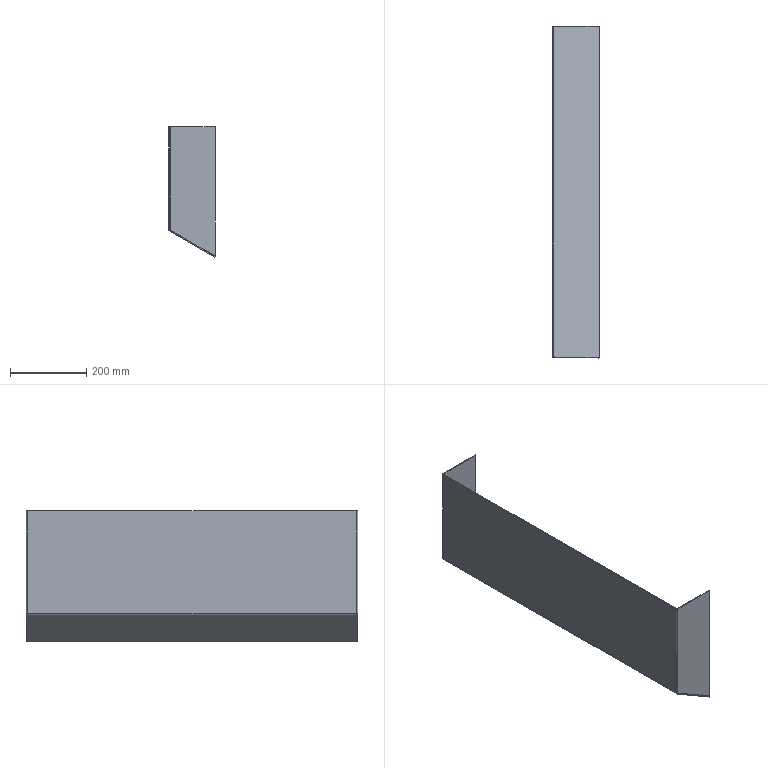Component | SolidWorks | AirInletVentAssembly-1_AirInletVentBaffle-5 | 1 solid | 32 faces | box 122 x 870 x 341.73 mm | volume 858235 mm3 | plane 24 | cylinder 6 | spline 2 | commonest cylinder face diameters 4 x3 8 x3 | material Plain Carbon Steel
STEP:
#1=CARTESIAN_POINT('',(96.744,7.148,50.154));
#2=VERTEX_POINT('',#1);
#3=CARTESIAN_POINT('',(96.744,41.085,50.154));
#4=VERTEX_POINT('',#3);
#5=CARTESIAN_POINT('',(96.744,6.99,50.154));
#6=DIRECTION('',(0.,1.,-0.));
#7=VECTOR('',#6,39.37);
#8=LINE('',#5,#7);
#9=EDGE_CURVE('',#2,#4,#8,.T.);
#10=ORIENTED_EDGE('',*,*,#9,.T.);
#11=CARTESIAN_POINT('',(96.744,41.085,60.767));
#12=VERTEX_POINT('',#11);
#13=CARTESIAN_POINT('',(96.744,41.085,60.767));
#14=DIRECTION('',(0.,-0.,-1.));
#15=VECTOR('',#14,39.37);
#16=LINE('',#13,#15);
#17=EDGE_CURVE('',#12,#4,#16,.T.);
#18=ORIENTED_EDGE('',*,*,#17,.F.);
#19=CARTESIAN_POINT('',(96.744,7.148,60.767));
#20=VERTEX_POINT('',#19);
#21=CARTESIAN_POINT('',(96.744,6.99,60.767));
#22=DIRECTION('',(0.,1.,-0.));
#23=VECTOR('',#22,39.37);
#24=LINE('',#21,#23);
#25=EDGE_CURVE('',#20,#12,#24,.T.);
#26=ORIENTED_EDGE('',*,*,#25,.F.);
#27=CARTESIAN_POINT('',(96.744,7.148,50.109));
#28=DIRECTION('',(-0.,0.,1.));
#29=VECTOR('',#28,39.37);
#30=LINE('',#27,#29);
#31=EDGE_CURVE('',#2,#20,#30,.T.);
#32=ORIENTED_EDGE('',*,*,#31,.F.);
#33=EDGE_LOOP('',(#10,#18,#26,#32));
#34=FACE_OUTER_BOUND('',#33,.T.);
#35=CARTESIAN_POINT('',(96.744,6.99,50.109));
#36=DIRECTION('',(1.,-0.,0.));
#37=DIRECTION('',(-0.,0.,1.));
#38=AXIS2_PLACEMENT_3D('',#35,#36,#37);
#39=PLANE('',#38);
#40=ADVANCED_FACE('',(#34),#39,.T.);
#41=CARTESIAN_POINT('',(96.665,41.085,60.767));
#42=VERTEX_POINT('',#41);
#43=CARTESIAN_POINT('',(96.665,41.085,50.154));
#44=VERTEX_POINT('',#43);
#45=CARTESIAN_POINT('',(96.665,41.085,60.767));
#46=DIRECTION('',(0.,-0.,-1.));
#47=VECTOR('',#46,39.37);
#48=LINE('',#45,#47);
#49=EDGE_CURVE('',#42,#44,#48,.T.);
#50=ORIENTED_EDGE('',*,*,#49,.T.);
#51=CARTESIAN_POINT('',(96.665,7.148,50.154));
#52=VERTEX_POINT('',#51);
#53=CARTESIAN_POINT('',(96.665,6.99,50.154));
#54=DIRECTION('',(0.,1.,-0.));
#55=VECTOR('',#54,39.37);
#56=LINE('',#53,#55);
#57=EDGE_CURVE('',#52,#44,#56,.T.);
#58=ORIENTED_EDGE('',*,*,#57,.F.);
#59=CARTESIAN_POINT('',(96.665,7.148,60.767));
#60=VERTEX_POINT('',#59);
#61=CARTESIAN_POINT('',(96.665,7.148,50.109));
#62=DIRECTION('',(-0.,0.,1.));
#63=VECTOR('',#62,39.37);
#64=LINE('',#61,#63);
#65=EDGE_CURVE('',#52,#60,#64,.T.);
#66=ORIENTED_EDGE('',*,*,#65,.T.);
#67=CARTESIAN_POINT('',(96.665,6.99,60.767));
#68=DIRECTION('',(0.,1.,-0.));
#69=VECTOR('',#68,39.37);
#70=LINE('',#67,#69);
#71=EDGE_CURVE('',#60,#42,#70,.T.);
#72=ORIENTED_EDGE('',*,*,#71,.T.);
#73=EDGE_LOOP('',(#50,#58,#66,#72));
#74=FACE_OUTER_BOUND('',#73,.T.);
#75=CARTESIAN_POINT('',(96.665,6.99,50.109));
#76=DIRECTION('',(1.,-0.,0.));
#77=DIRECTION('',(-0.,0.,1.));
#78=AXIS2_PLACEMENT_3D('',#75,#76,#77);
#79=PLANE('',#78);
#80=ADVANCED_FACE('',(#74),#79,.F.);
#81=ORIENTED_EDGE('',*,*,#25,.T.);
#82=CARTESIAN_POINT('',(96.744,41.085,60.767));
#83=DIRECTION('',(-1.,0.,-0.));
#84=VECTOR('',#83,39.37);
#85=LINE('',#82,#84);
#86=EDGE_CURVE('',#12,#42,#85,.T.);
#87=ORIENTED_EDGE('',*,*,#86,.T.);
#88=ORIENTED_EDGE('',*,*,#71,.F.);
#89=CARTESIAN_POINT('',(96.744,7.148,60.767));
#90=DIRECTION('',(-1.,0.,-0.));
#91=VECTOR('',#90,39.37);
#92=LINE('',#89,#91);
#93=EDGE_CURVE('',#20,#60,#92,.T.);
#94=ORIENTED_EDGE('',*,*,#93,.F.);
#95=EDGE_LOOP('',(#81,#87,#88,#94));
#96=FACE_OUTER_BOUND('',#95,.T.);
#97=CARTESIAN_POINT('',(96.665,6.99,60.767));
#98=DIRECTION('',(-0.,0.,1.));
#99=DIRECTION('',(-0.,-1.,0.));
#100=AXIS2_PLACEMENT_3D('',#97,#98,#99);
#101=PLANE('',#100);
#102=ADVANCED_FACE('',(#96),#101,.T.);
#103=CARTESIAN_POINT('',(96.783,6.99,50.086));
#104=VERTEX_POINT('',#103);
#105=CARTESIAN_POINT('',(96.744,6.99,50.018));
#106=VERTEX_POINT('',#105);
#107=CARTESIAN_POINT('',(96.783,6.99,50.086));
#108=DIRECTION('',(-0.5,-0.,-0.866));
#109=VECTOR('',#108,39.37);
#110=LINE('',#107,#109);
#111=EDGE_CURVE('',#104,#106,#110,.T.);
#112=ORIENTED_EDGE('',*,*,#111,.F.);
#113=CARTESIAN_POINT('',(96.744,6.99,50.154));
#114=VERTEX_POINT('',#113);
#115=CARTESIAN_POINT('',(96.822,6.99,50.154));
#116=DIRECTION('',(-0.,-1.,0.));
#117=DIRECTION('',(-1.,0.,0.));
#118=AXIS2_PLACEMENT_3D('',#115,#116,#117);
#119=CIRCLE('',#118,0.07874);
#120=EDGE_CURVE('',#114,#104,#119,.T.);
#121=ORIENTED_EDGE('',*,*,#120,.F.);
#122=CARTESIAN_POINT('',(96.665,6.99,50.154));
#123=VERTEX_POINT('',#122);
#124=CARTESIAN_POINT('',(96.665,6.99,50.154));
#125=DIRECTION('',(1.,-0.,0.));
#126=VECTOR('',#125,39.37);
#127=LINE('',#124,#126);
#128=EDGE_CURVE('',#123,#114,#127,.T.);
#129=ORIENTED_EDGE('',*,*,#128,.F.);
#130=CARTESIAN_POINT('',(96.822,6.99,50.154));
#131=DIRECTION('',(-0.,-1.,0.));
#132=DIRECTION('',(1.,-0.,0.));
#133=AXIS2_PLACEMENT_3D('',#130,#131,#132);
#134=CIRCLE('',#133,0.1575);
#135=EDGE_CURVE('',#123,#106,#134,.T.);
#136=ORIENTED_EDGE('',*,*,#135,.T.);
#137=EDGE_LOOP('',(#112,#121,#129,#136));
#138=FACE_OUTER_BOUND('',#137,.T.);
#139=CARTESIAN_POINT('',(96.783,6.99,50.086));
#140=DIRECTION('',(-0.,-1.,0.));
#141=DIRECTION('',(1.,-0.,0.));
#142=AXIS2_PLACEMENT_3D('',#139,#140,#141);
#143=PLANE('',#142);
#144=ADVANCED_FACE('',(#138),#143,.T.);
#145=CARTESIAN_POINT('',(101.468,6.99,47.381));
#146=VERTEX_POINT('',#145);
#147=CARTESIAN_POINT('',(96.744,6.99,50.109));
#148=DIRECTION('',(0.866,-0.,-0.5));
#149=VECTOR('',#148,39.37);
#150=LINE('',#147,#149);
#151=EDGE_CURVE('',#104,#146,#150,.T.);
#152=ORIENTED_EDGE('',*,*,#151,.F.);
#153=ORIENTED_EDGE('',*,*,#111,.T.);
#154=CARTESIAN_POINT('',(101.429,6.99,47.313));
#155=VERTEX_POINT('',#154);
#156=CARTESIAN_POINT('',(96.704,6.99,50.04));
#157=DIRECTION('',(0.866,-0.,-0.5));
#158=VECTOR('',#157,39.37);
#159=LINE('',#156,#158);
#160=EDGE_CURVE('',#106,#155,#159,.T.);
#161=ORIENTED_EDGE('',*,*,#160,.T.);
#162=CARTESIAN_POINT('',(101.468,6.99,47.381));
#163=DIRECTION('',(-0.5,-0.,-0.866));
#164=VECTOR('',#163,39.37);
#165=LINE('',#162,#164);
#166=EDGE_CURVE('',#146,#155,#165,.T.);
#167=ORIENTED_EDGE('',*,*,#166,.F.);
#168=EDGE_LOOP('',(#152,#153,#161,#167));
#169=FACE_OUTER_BOUND('',#168,.T.);
#170=CARTESIAN_POINT('',(96.665,6.99,50.154));
#171=DIRECTION('',(-0.,-1.,0.));
#172=DIRECTION('',(1.,-0.,0.));
#173=AXIS2_PLACEMENT_3D('',#170,#171,#172);
#174=PLANE('',#173);
#175=ADVANCED_FACE('',(#169),#174,.T.);
#176=CARTESIAN_POINT('',(96.744,41.242,50.154));
#177=VERTEX_POINT('',#176);
#178=CARTESIAN_POINT('',(96.665,41.242,50.154));
#179=VERTEX_POINT('',#178);
#180=CARTESIAN_POINT('',(96.744,41.242,50.154));
#181=DIRECTION('',(-1.,0.,-0.));
#182=VECTOR('',#181,39.37);
#183=LINE('',#180,#182);
#184=EDGE_CURVE('',#177,#179,#183,.T.);
#185=ORIENTED_EDGE('',*,*,#184,.F.);
#186=CARTESIAN_POINT('',(96.783,41.242,50.086));
#187=VERTEX_POINT('',#186);
#188=CARTESIAN_POINT('',(96.822,41.242,50.154));
#189=DIRECTION('',(-0.,-1.,0.));
#190=DIRECTION('',(-1.,0.,0.));
#191=AXIS2_PLACEMENT_3D('',#188,#189,#190);
#192=CIRCLE('',#191,0.07874);
#193=EDGE_CURVE('',#177,#187,#192,.T.);
#194=ORIENTED_EDGE('',*,*,#193,.T.);
#195=CARTESIAN_POINT('',(96.744,41.242,50.018));
#196=VERTEX_POINT('',#195);
#197=CARTESIAN_POINT('',(96.744,41.242,50.018));
#198=DIRECTION('',(0.5,0.,0.866));
#199=VECTOR('',#198,39.37);
#200=LINE('',#197,#199);
#201=EDGE_CURVE('',#196,#187,#200,.T.);
#202=ORIENTED_EDGE('',*,*,#201,.F.);
#203=CARTESIAN_POINT('',(96.822,41.242,50.154));
#204=DIRECTION('',(-0.,-1.,0.));
#205=DIRECTION('',(1.,0.,0.));
#206=AXIS2_PLACEMENT_3D('',#203,#204,#205);
#207=CIRCLE('',#206,0.1575);
#208=EDGE_CURVE('',#179,#196,#207,.T.);
#209=ORIENTED_EDGE('',*,*,#208,.F.);
#210=EDGE_LOOP('',(#185,#194,#202,#209));
#211=FACE_OUTER_BOUND('',#210,.T.);
#212=CARTESIAN_POINT('',(96.744,41.242,50.154));
#213=DIRECTION('',(0.,1.,-0.));
#214=DIRECTION('',(-1.,0.,-0.));
#215=AXIS2_PLACEMENT_3D('',#212,#213,#214);
#216=PLANE('',#215);
#217=ADVANCED_FACE('',(#211),#216,.T.);
#218=CARTESIAN_POINT('',(101.429,41.242,47.313));
#219=VERTEX_POINT('',#218);
#220=CARTESIAN_POINT('',(96.704,41.242,50.04));
#221=DIRECTION('',(0.866,-0.,-0.5));
#222=VECTOR('',#221,39.37);
#223=LINE('',#220,#222);
#224=EDGE_CURVE('',#196,#219,#223,.T.);
#225=ORIENTED_EDGE('',*,*,#224,.T.);
#226=CARTESIAN_POINT('',(101.429,6.99,47.313));
#227=DIRECTION('',(0.,1.,-0.));
#228=VECTOR('',#227,39.37);
#229=LINE('',#226,#228);
#230=EDGE_CURVE('',#155,#219,#229,.T.);
#231=ORIENTED_EDGE('',*,*,#230,.F.);
#232=ORIENTED_EDGE('',*,*,#160,.F.);
#233=CARTESIAN_POINT('',(96.744,6.99,50.018));
#234=DIRECTION('',(0.,1.,-0.));
#235=VECTOR('',#234,39.37);
#236=LINE('',#233,#235);
#237=EDGE_CURVE('',#106,#196,#236,.T.);
#238=ORIENTED_EDGE('',*,*,#237,.T.);
#239=EDGE_LOOP('',(#225,#231,#232,#238));
#240=FACE_OUTER_BOUND('',#239,.T.);
#241=CARTESIAN_POINT('',(96.704,6.99,50.04));
#242=DIRECTION('',(0.5,0.,0.866));
#243=DIRECTION('',(-0.866,0.,0.5));
#244=AXIS2_PLACEMENT_3D('',#241,#242,#243);
#245=PLANE('',#244);
#246=ADVANCED_FACE('',(#240),#245,.F.);
#247=CARTESIAN_POINT('',(101.468,41.242,47.381));
#248=VERTEX_POINT('',#247);
#249=CARTESIAN_POINT('',(101.468,41.242,47.381));
#250=DIRECTION('',(-0.5,-0.,-0.866));
#251=VECTOR('',#250,39.37);
#252=LINE('',#249,#251);
#253=EDGE_CURVE('',#248,#219,#252,.T.);
#254=ORIENTED_EDGE('',*,*,#253,.F.);
#255=CARTESIAN_POINT('',(101.468,6.99,47.381));
#256=DIRECTION('',(0.,1.,-0.));
#257=VECTOR('',#256,39.37);
#258=LINE('',#255,#257);
#259=EDGE_CURVE('',#146,#248,#258,.T.);
#260=ORIENTED_EDGE('',*,*,#259,.F.);
#261=ORIENTED_EDGE('',*,*,#166,.T.);
#262=ORIENTED_EDGE('',*,*,#230,.T.);
#263=EDGE_LOOP('',(#254,#260,#261,#262));
#264=FACE_OUTER_BOUND('',#263,.T.);
#265=CARTESIAN_POINT('',(101.468,6.99,47.381));
#266=DIRECTION('',(0.866,-0.,-0.5));
#267=DIRECTION('',(0.5,0.,0.866));
#268=AXIS2_PLACEMENT_3D('',#265,#266,#267);
#269=PLANE('',#268);
#270=ADVANCED_FACE('',(#264),#269,.T.);
#271=CARTESIAN_POINT('',(96.744,41.242,50.109));
#272=DIRECTION('',(0.866,-0.,-0.5));
#273=VECTOR('',#272,39.37);
#274=LINE('',#271,#273);
#275=EDGE_CURVE('',#187,#248,#274,.T.);
#276=ORIENTED_EDGE('',*,*,#275,.F.);
#277=CARTESIAN_POINT('',(96.783,6.99,50.086));
#278=DIRECTION('',(0.,1.,-0.));
#279=VECTOR('',#278,39.37);
#280=LINE('',#277,#279);
#281=EDGE_CURVE('',#104,#187,#280,.T.);
#282=ORIENTED_EDGE('',*,*,#281,.F.);
#283=ORIENTED_EDGE('',*,*,#151,.T.);
#284=ORIENTED_EDGE('',*,*,#259,.T.);
#285=EDGE_LOOP('',(#276,#282,#283,#284));
#286=FACE_OUTER_BOUND('',#285,.T.);
#287=CARTESIAN_POINT('',(96.744,6.99,50.109));
#288=DIRECTION('',(0.5,0.,0.866));
#289=DIRECTION('',(-0.866,0.,0.5));
#290=AXIS2_PLACEMENT_3D('',#287,#288,#289);
#291=PLANE('',#290);
#292=ADVANCED_FACE('',(#286),#291,.T.);
#293=ORIENTED_EDGE('',*,*,#193,.F.);
#294=CARTESIAN_POINT('',(96.744,41.085,50.154));
#295=DIRECTION('',(0.,1.,-0.));
#296=VECTOR('',#295,39.37);
#297=LINE('',#294,#296);
#298=EDGE_CURVE('',#4,#177,#297,.T.);
#299=ORIENTED_EDGE('',*,*,#298,.F.);
#300=ORIENTED_EDGE('',*,*,#9,.F.);
#301=CARTESIAN_POINT('',(96.744,6.99,50.154));
#302=DIRECTION('',(0.,1.,-0.));
#303=VECTOR('',#302,39.37);
#304=LINE('',#301,#303);
#305=EDGE_CURVE('',#114,#2,#304,.T.);
#306=ORIENTED_EDGE('',*,*,#305,.F.);
#307=ORIENTED_EDGE('',*,*,#120,.T.);
#308=ORIENTED_EDGE('',*,*,#281,.T.);
#309=EDGE_LOOP('',(#293,#299,#300,#306,#307,#308));
#310=FACE_OUTER_BOUND('',#309,.T.);
#311=CARTESIAN_POINT('',(96.822,6.99,50.154));
#312=DIRECTION('',(0.,1.,-0.));
#313=DIRECTION('',(-1.,0.,0.));
#314=AXIS2_PLACEMENT_3D('',#311,#312,#313);
#315=CYLINDRICAL_SURFACE('',#314,0.07874);
#316=ADVANCED_FACE('',(#310),#315,.F.);
#317=ORIENTED_EDGE('',*,*,#208,.T.);
#318=ORIENTED_EDGE('',*,*,#237,.F.);
#319=ORIENTED_EDGE('',*,*,#135,.F.);
#320=CARTESIAN_POINT('',(96.665,6.99,50.154));
#321=DIRECTION('',(0.,1.,-0.));
#322=VECTOR('',#321,39.37);
#323=LINE('',#320,#322);
#324=EDGE_CURVE('',#123,#52,#323,.T.);
#325=ORIENTED_EDGE('',*,*,#324,.T.);
#326=ORIENTED_EDGE('',*,*,#57,.T.);
#327=CARTESIAN_POINT('',(96.665,6.99,50.154));
#328=DIRECTION('',(0.,1.,-0.));
#329=VECTOR('',#328,39.37);
#330=LINE('',#327,#329);
#331=EDGE_CURVE('',#44,#179,#330,.T.);
#332=ORIENTED_EDGE('',*,*,#331,.T.);
#333=EDGE_LOOP('',(#317,#318,#319,#325,#326,#332));
#334=FACE_OUTER_BOUND('',#333,.T.);
#335=CARTESIAN_POINT('',(96.822,6.99,50.154));
#336=DIRECTION('',(0.,1.,-0.));
#337=DIRECTION('',(-1.,0.,0.));
#338=AXIS2_PLACEMENT_3D('',#335,#336,#337);
#339=CYLINDRICAL_SURFACE('',#338,0.1575);
#340=ADVANCED_FACE('',(#334),#339,.T.);
#341=ORIENTED_EDGE('',*,*,#224,.F.);
#342=ORIENTED_EDGE('',*,*,#201,.T.);
#343=ORIENTED_EDGE('',*,*,#275,.T.);
#344=ORIENTED_EDGE('',*,*,#253,.T.);
#345=EDGE_LOOP('',(#341,#342,#343,#344));
#346=FACE_OUTER_BOUND('',#345,.T.);
#347=CARTESIAN_POINT('',(96.822,41.242,50.154));
#348=DIRECTION('',(0.,1.,-0.));
#349=DIRECTION('',(-1.,0.,-0.));
#350=AXIS2_PLACEMENT_3D('',#347,#348,#349);
#351=PLANE('',#350);
#352=ADVANCED_FACE('',(#346),#351,.T.);
#353=CARTESIAN_POINT('',(96.744,7.148,50.154));
#354=DIRECTION('',(-1.,0.,-0.));
#355=VECTOR('',#354,39.37);
#356=LINE('',#353,#355);
#357=EDGE_CURVE('',#2,#52,#356,.T.);
#358=ORIENTED_EDGE('',*,*,#357,.T.);
#359=ORIENTED_EDGE('',*,*,#324,.F.);
#360=ORIENTED_EDGE('',*,*,#128,.T.);
#361=ORIENTED_EDGE('',*,*,#305,.T.);
#362=EDGE_LOOP('',(#358,#359,#360,#361));
#363=FACE_OUTER_BOUND('',#362,.T.);
#364=CARTESIAN_POINT('',(96.744,6.99,50.154));
#365=DIRECTION('',(-0.,0.,1.));
#366=DIRECTION('',(-0.,-1.,0.));
#367=AXIS2_PLACEMENT_3D('',#364,#365,#366);
#368=PLANE('',#367);
#369=ADVANCED_FACE('',(#363),#368,.T.);
#370=CARTESIAN_POINT('',(96.822,7.069,60.767));
#371=VERTEX_POINT('',#370);
#372=CARTESIAN_POINT('',(96.822,6.99,60.767));
#373=VERTEX_POINT('',#372);
#374=CARTESIAN_POINT('',(96.822,6.99,60.767));
#375=DIRECTION('',(-0.,-1.,0.));
#376=VECTOR('',#375,39.37);
#377=LINE('',#374,#376);
#378=EDGE_CURVE('',#371,#373,#377,.T.);
#379=ORIENTED_EDGE('',*,*,#378,.F.);
#380=CARTESIAN_POINT('',(96.822,7.148,60.767));
#381=DIRECTION('',(-0.,0.,1.));
#382=DIRECTION('',(0.,1.,0.));
#383=AXIS2_PLACEMENT_3D('',#380,#381,#382);
#384=CIRCLE('',#383,0.07874);
#385=EDGE_CURVE('',#20,#371,#384,.T.);
#386=ORIENTED_EDGE('',*,*,#385,.F.);
#387=ORIENTED_EDGE('',*,*,#93,.T.);
#388=CARTESIAN_POINT('',(96.822,7.148,60.767));
#389=DIRECTION('',(-0.,0.,1.));
#390=DIRECTION('',(0.,1.,0.));
#391=AXIS2_PLACEMENT_3D('',#388,#389,#390);
#392=CIRCLE('',#391,0.1575);
#393=EDGE_CURVE('',#60,#373,#392,.T.);
#394=ORIENTED_EDGE('',*,*,#393,.T.);
#395=EDGE_LOOP('',(#379,#386,#387,#394));
#396=FACE_OUTER_BOUND('',#395,.T.);
#397=CARTESIAN_POINT('',(96.822,7.148,60.767));
#398=DIRECTION('',(-0.,0.,1.));
#399=DIRECTION('',(-0.,-1.,0.));
#400=AXIS2_PLACEMENT_3D('',#397,#398,#399);
#401=PLANE('',#400);
#402=ADVANCED_FACE('',(#396),#401,.T.);
#403=CARTESIAN_POINT('',(96.822,7.069,50.109));
#404=VERTEX_POINT('',#403);
#405=CARTESIAN_POINT('',(96.822,7.069,50.109));
#406=CARTESIAN_POINT('',(96.817,7.069,50.111));
#407=CARTESIAN_POINT('',(96.812,7.069,50.112));
#408=CARTESIAN_POINT('',(96.802,7.071,50.116));
#409=CARTESIAN_POINT('',(96.797,7.073,50.118));
#410=CARTESIAN_POINT('',(96.787,7.077,50.122));
#411=CARTESIAN_POINT('',(96.783,7.079,50.124));
#412=CARTESIAN_POINT('',(96.774,7.085,50.128));
#413=CARTESIAN_POINT('',(96.77,7.088,50.13));
#414=CARTESIAN_POINT('',(96.763,7.096,50.133));
#415=CARTESIAN_POINT('',(96.76,7.1,50.135));
#416=CARTESIAN_POINT('',(96.754,7.108,50.139));
#417=CARTESIAN_POINT('',(96.752,7.113,50.141));
#418=CARTESIAN_POINT('',(96.748,7.122,50.145));
#419=CARTESIAN_POINT('',(96.746,7.127,50.147));
#420=CARTESIAN_POINT('',(96.744,7.137,50.15));
#421=CARTESIAN_POINT('',(96.744,7.142,50.152));
#422=CARTESIAN_POINT('',(96.744,7.148,50.154));
#423=B_SPLINE_CURVE_WITH_KNOTS('',3,(#405,#406,#407,#408,#409,#410,#411,#412,#413,#414,#415,#416,#417,#418,#419,#420,#421,#422),.UNSPECIFIED.,.F.,.F.,(4,2,2,2,2,2,2,2,4),(0.,0.0004161,0.0008322,0.001248,0.001664,0.002081,0.002497,0.002913,0.003329),.UNSPECIFIED.);
#424=EDGE_CURVE('',#404,#2,#423,.T.);
#425=ORIENTED_EDGE('',*,*,#424,.F.);
#426=CARTESIAN_POINT('',(96.822,6.99,50.109));
#427=VERTEX_POINT('',#426);
#428=CARTESIAN_POINT('',(96.822,7.069,50.109));
#429=DIRECTION('',(-0.,-1.,0.));
#430=VECTOR('',#429,39.37);
#431=LINE('',#428,#430);
#432=EDGE_CURVE('',#404,#427,#431,.T.);
#433=ORIENTED_EDGE('',*,*,#432,.T.);
#434=CARTESIAN_POINT('',(96.822,6.99,50.109));
#435=CARTESIAN_POINT('',(96.812,6.99,50.111));
#436=CARTESIAN_POINT('',(96.802,6.991,50.112));
#437=CARTESIAN_POINT('',(96.782,6.995,50.116));
#438=CARTESIAN_POINT('',(96.772,6.998,50.118));
#439=CARTESIAN_POINT('',(96.753,7.006,50.122));
#440=CARTESIAN_POINT('',(96.743,7.011,50.124));
#441=CARTESIAN_POINT('',(96.726,7.022,50.128));
#442=CARTESIAN_POINT('',(96.718,7.029,50.13));
#443=CARTESIAN_POINT('',(96.704,7.043,50.133));
#444=CARTESIAN_POINT('',(96.697,7.051,50.135));
#445=CARTESIAN_POINT('',(96.686,7.069,50.139));
#446=CARTESIAN_POINT('',(96.681,7.078,50.141));
#447=CARTESIAN_POINT('',(96.669,7.106,50.147));
#448=CARTESIAN_POINT('',(96.665,7.127,50.15));
#449=CARTESIAN_POINT('',(96.665,7.148,50.154));
#450=B_SPLINE_CURVE_WITH_KNOTS('',3,(#434,#435,#436,#437,#438,#439,#440,#441,#442,#443,#444,#445,#446,#447,#448,#449),.UNSPECIFIED.,.F.,.F.,(4,2,2,2,2,2,2,4),(0.,0.0007941,0.001588,0.002382,0.003177,0.003971,0.004765,0.006353),.UNSPECIFIED.);
#451=EDGE_CURVE('',#427,#52,#450,.T.);
#452=ORIENTED_EDGE('',*,*,#451,.T.);
#453=ORIENTED_EDGE('',*,*,#357,.F.);
#454=EDGE_LOOP('',(#425,#433,#452,#453));
#455=FACE_OUTER_BOUND('',#454,.T.);
#456=CARTESIAN_POINT('',(96.822,6.989,50.109));
#457=CARTESIAN_POINT('',(96.802,6.989,50.112));
#458=CARTESIAN_POINT('',(96.781,6.993,50.116));
#459=CARTESIAN_POINT('',(96.743,7.009,50.124));
#460=CARTESIAN_POINT('',(96.725,7.021,50.128));
#461=CARTESIAN_POINT('',(96.696,7.05,50.135));
#462=CARTESIAN_POINT('',(96.684,7.068,50.139));
#463=CARTESIAN_POINT('',(96.668,7.106,50.147));
#464=CARTESIAN_POINT('',(96.664,7.127,50.15));
#465=CARTESIAN_POINT('',(96.664,7.148,50.154));
#466=CARTESIAN_POINT('',(96.822,6.99,50.109));
#467=CARTESIAN_POINT('',(96.802,6.99,50.112));
#468=CARTESIAN_POINT('',(96.781,6.994,50.116));
#469=CARTESIAN_POINT('',(96.743,7.01,50.124));
#470=CARTESIAN_POINT('',(96.726,7.022,50.128));
#471=CARTESIAN_POINT('',(96.696,7.051,50.135));
#472=CARTESIAN_POINT('',(96.685,7.068,50.139));
#473=CARTESIAN_POINT('',(96.669,7.106,50.147));
#474=CARTESIAN_POINT('',(96.665,7.127,50.15));
#475=CARTESIAN_POINT('',(96.665,7.148,50.154));
#476=CARTESIAN_POINT('',(96.822,7.069,50.109));
#477=CARTESIAN_POINT('',(96.812,7.069,50.112));
#478=CARTESIAN_POINT('',(96.802,7.071,50.116));
#479=CARTESIAN_POINT('',(96.783,7.079,50.124));
#480=CARTESIAN_POINT('',(96.774,7.085,50.128));
#481=CARTESIAN_POINT('',(96.759,7.099,50.135));
#482=CARTESIAN_POINT('',(96.754,7.108,50.139));
#483=CARTESIAN_POINT('',(96.746,7.127,50.147));
#484=CARTESIAN_POINT('',(96.744,7.137,50.15));
#485=CARTESIAN_POINT('',(96.744,7.148,50.154));
#486=CARTESIAN_POINT('',(96.822,7.07,50.109));
#487=CARTESIAN_POINT('',(96.812,7.07,50.112));
#488=CARTESIAN_POINT('',(96.802,7.072,50.116));
#489=CARTESIAN_POINT('',(96.783,7.079,50.124));
#490=CARTESIAN_POINT('',(96.774,7.085,50.128));
#491=CARTESIAN_POINT('',(96.76,7.1,50.135));
#492=CARTESIAN_POINT('',(96.754,7.108,50.139));
#493=CARTESIAN_POINT('',(96.746,7.127,50.147));
#494=CARTESIAN_POINT('',(96.744,7.137,50.15));
#495=CARTESIAN_POINT('',(96.744,7.148,50.154));
#496=B_SPLINE_SURFACE_WITH_KNOTS('',1,3,((#456,#457,#458,#459,#460,#461,#462,#463,#464,#465),(#466,#467,#468,#469,#470,#471,#472,#473,#474,#475),(#476,#477,#478,#479,#480,#481,#482,#483,#484,#485),(#486,#487,#488,#489,#490,#491,#492,#493,#494,#495)),.UNSPECIFIED.,.F.,.F.,.F.,(2,1,1,2),(4,2,2,2,4),(-0.01,0.,1.,1.01),(0.,0.25,0.5,0.75,1.),.UNSPECIFIED.);
#497=ADVANCED_FACE('',(#455),#496,.F.);
#498=ORIENTED_EDGE('',*,*,#65,.F.);
#499=ORIENTED_EDGE('',*,*,#451,.F.);
#500=CARTESIAN_POINT('',(96.822,6.99,60.767));
#501=DIRECTION('',(-0.,0.,1.));
#502=VECTOR('',#501,39.37);
#503=LINE('',#500,#502);
#504=EDGE_CURVE('',#427,#373,#503,.T.);
#505=ORIENTED_EDGE('',*,*,#504,.T.);
#506=ORIENTED_EDGE('',*,*,#393,.F.);
#507=EDGE_LOOP('',(#498,#499,#505,#506));
#508=FACE_OUTER_BOUND('',#507,.T.);
#509=CARTESIAN_POINT('',(96.822,7.148,50.109));
#510=DIRECTION('',(0.,-0.,-1.));
#511=DIRECTION('',(0.,-1.,0.));
#512=AXIS2_PLACEMENT_3D('',#509,#510,#511);
#513=CYLINDRICAL_SURFACE('',#512,0.1575);
#514=ADVANCED_FACE('',(#508),#513,.T.);
#515=ORIENTED_EDGE('',*,*,#31,.T.);
#516=ORIENTED_EDGE('',*,*,#385,.T.);
#517=CARTESIAN_POINT('',(96.822,7.069,60.767));
#518=DIRECTION('',(0.,-0.,-1.));
#519=VECTOR('',#518,39.37);
#520=LINE('',#517,#519);
#521=EDGE_CURVE('',#371,#404,#520,.T.);
#522=ORIENTED_EDGE('',*,*,#521,.T.);
#523=ORIENTED_EDGE('',*,*,#424,.T.);
#524=EDGE_LOOP('',(#515,#516,#522,#523));
#525=FACE_OUTER_BOUND('',#524,.T.);
#526=CARTESIAN_POINT('',(96.822,7.148,50.109));
#527=DIRECTION('',(0.,-0.,-1.));
#528=DIRECTION('',(0.,-1.,0.));
#529=AXIS2_PLACEMENT_3D('',#526,#527,#528);
#530=CYLINDRICAL_SURFACE('',#529,0.07874);
#531=ADVANCED_FACE('',(#525),#530,.F.);
#532=ORIENTED_EDGE('',*,*,#378,.T.);
#533=CARTESIAN_POINT('',(101.468,6.99,60.767));
#534=VERTEX_POINT('',#533);
#535=CARTESIAN_POINT('',(96.744,6.99,60.767));
#536=DIRECTION('',(-1.,0.,-0.));
#537=VECTOR('',#536,39.37);
#538=LINE('',#535,#537);
#539=EDGE_CURVE('',#534,#373,#538,.T.);
#540=ORIENTED_EDGE('',*,*,#539,.F.);
#541=CARTESIAN_POINT('',(101.468,7.069,60.767));
#542=VERTEX_POINT('',#541);
#543=CARTESIAN_POINT('',(101.468,6.99,60.767));
#544=DIRECTION('',(0.,1.,-0.));
#545=VECTOR('',#544,39.37);
#546=LINE('',#543,#545);
#547=EDGE_CURVE('',#534,#542,#546,.T.);
#548=ORIENTED_EDGE('',*,*,#547,.T.);
#549=CARTESIAN_POINT('',(96.744,7.069,60.767));
#550=DIRECTION('',(-1.,0.,-0.));
#551=VECTOR('',#550,39.37);
#552=LINE('',#549,#551);
#553=EDGE_CURVE('',#542,#371,#552,.T.);
#554=ORIENTED_EDGE('',*,*,#553,.T.);
#555=EDGE_LOOP('',(#532,#540,#548,#554));
#556=FACE_OUTER_BOUND('',#555,.T.);
#557=CARTESIAN_POINT('',(96.744,6.99,60.767));
#558=DIRECTION('',(0.,-0.,-1.));
#559=DIRECTION('',(0.,1.,-0.));
#560=AXIS2_PLACEMENT_3D('',#557,#558,#559);
#561=PLANE('',#560);
#562=ADVANCED_FACE('',(#556),#561,.F.);
#563=ORIENTED_EDGE('',*,*,#432,.F.);
#564=CARTESIAN_POINT('',(101.468,7.069,47.427));
#565=VERTEX_POINT('',#564);
#566=CARTESIAN_POINT('',(96.744,7.069,50.154));
#567=DIRECTION('',(0.866,-0.,-0.5));
#568=VECTOR('',#567,39.37);
#569=LINE('',#566,#568);
#570=EDGE_CURVE('',#404,#565,#569,.T.);
#571=ORIENTED_EDGE('',*,*,#570,.T.);
#572=CARTESIAN_POINT('',(101.468,6.99,47.427));
#573=VERTEX_POINT('',#572);
#574=CARTESIAN_POINT('',(101.468,6.99,47.427));
#575=DIRECTION('',(0.,1.,-0.));
#576=VECTOR('',#575,39.37);
#577=LINE('',#574,#576);
#578=EDGE_CURVE('',#573,#565,#577,.T.);
#579=ORIENTED_EDGE('',*,*,#578,.F.);
#580=CARTESIAN_POINT('',(96.763,6.99,50.143));
#581=DIRECTION('',(0.866,-0.,-0.5));
#582=VECTOR('',#581,39.37);
#583=LINE('',#580,#582);
#584=EDGE_CURVE('',#427,#573,#583,.T.);
#585=ORIENTED_EDGE('',*,*,#584,.F.);
#586=EDGE_LOOP('',(#563,#571,#579,#585));
#587=FACE_OUTER_BOUND('',#586,.T.);
#588=CARTESIAN_POINT('',(96.744,6.99,50.154));
#589=DIRECTION('',(0.5,-0.,0.866));
#590=DIRECTION('',(-0.866,0.,0.5));
#591=AXIS2_PLACEMENT_3D('',#588,#589,#590);
#592=PLANE('',#591);
#593=ADVANCED_FACE('',(#587),#592,.F.);
#594=ORIENTED_EDGE('',*,*,#504,.F.);
#595=ORIENTED_EDGE('',*,*,#584,.T.);
#596=CARTESIAN_POINT('',(101.468,6.99,50.109));
#597=DIRECTION('',(-0.,0.,1.));
#598=VECTOR('',#597,39.37);
#599=LINE('',#596,#598);
#600=EDGE_CURVE('',#573,#534,#599,.T.);
#601=ORIENTED_EDGE('',*,*,#600,.T.);
#602=ORIENTED_EDGE('',*,*,#539,.T.);
#603=EDGE_LOOP('',(#594,#595,#601,#602));
#604=FACE_OUTER_BOUND('',#603,.T.);
#605=CARTESIAN_POINT('',(96.744,6.99,50.109));
#606=DIRECTION('',(0.,1.,-0.));
#607=DIRECTION('',(-1.,0.,-0.));
#608=AXIS2_PLACEMENT_3D('',#605,#606,#607);
#609=PLANE('',#608);
#610=ADVANCED_FACE('',(#604),#609,.F.);
#611=ORIENTED_EDGE('',*,*,#570,.F.);
#612=ORIENTED_EDGE('',*,*,#521,.F.);
#613=ORIENTED_EDGE('',*,*,#553,.F.);
#614=CARTESIAN_POINT('',(101.468,7.069,60.767));
#615=DIRECTION('',(-0.,0.,1.));
#616=VECTOR('',#615,39.37);
#617=LINE('',#614,#616);
#618=EDGE_CURVE('',#565,#542,#617,.T.);
#619=ORIENTED_EDGE('',*,*,#618,.F.);
#620=EDGE_LOOP('',(#611,#612,#613,#619));
#621=FACE_OUTER_BOUND('',#620,.T.);
#622=CARTESIAN_POINT('',(96.744,7.069,50.109));
#623=DIRECTION('',(0.,1.,-0.));
#624=DIRECTION('',(-1.,0.,-0.));
#625=AXIS2_PLACEMENT_3D('',#622,#623,#624);
#626=PLANE('',#625);
#627=ADVANCED_FACE('',(#621),#626,.T.);
#628=ORIENTED_EDGE('',*,*,#618,.T.);
#629=ORIENTED_EDGE('',*,*,#547,.F.);
#630=ORIENTED_EDGE('',*,*,#600,.F.);
#631=ORIENTED_EDGE('',*,*,#578,.T.);
#632=EDGE_LOOP('',(#628,#629,#630,#631));
#633=FACE_OUTER_BOUND('',#632,.T.);
#634=CARTESIAN_POINT('',(101.468,6.99,60.767));
#635=DIRECTION('',(-1.,0.,-0.));
#636=DIRECTION('',(-0.,-1.,0.));
#637=AXIS2_PLACEMENT_3D('',#634,#635,#636);
#638=PLANE('',#637);
#639=ADVANCED_FACE('',(#633),#638,.F.);
#640=ORIENTED_EDGE('',*,*,#184,.T.);
#641=ORIENTED_EDGE('',*,*,#331,.F.);
#642=CARTESIAN_POINT('',(96.744,41.085,50.154));
#643=DIRECTION('',(-1.,0.,-0.));
#644=VECTOR('',#643,39.37);
#645=LINE('',#642,#644);
#646=EDGE_CURVE('',#4,#44,#645,.T.);
#647=ORIENTED_EDGE('',*,*,#646,.F.);
#648=ORIENTED_EDGE('',*,*,#298,.T.);
#649=EDGE_LOOP('',(#640,#641,#647,#648));
#650=FACE_OUTER_BOUND('',#649,.T.);
#651=CARTESIAN_POINT('',(96.744,41.085,50.154));
#652=DIRECTION('',(-0.,0.,1.));
#653=DIRECTION('',(-0.,-1.,0.));
#654=AXIS2_PLACEMENT_3D('',#651,#652,#653);
#655=PLANE('',#654);
#656=ADVANCED_FACE('',(#650),#655,.T.);
#657=CARTESIAN_POINT('',(96.822,41.163,50.109));
#658=VERTEX_POINT('',#657);
#659=CARTESIAN_POINT('',(96.822,41.242,50.109));
#660=VERTEX_POINT('',#659);
#661=CARTESIAN_POINT('',(96.822,41.242,50.109));
#662=DIRECTION('',(0.,1.,-0.));
#663=VECTOR('',#662,39.37);
#664=LINE('',#661,#663);
#665=EDGE_CURVE('',#658,#660,#664,.T.);
#666=ORIENTED_EDGE('',*,*,#665,.F.);
#667=CARTESIAN_POINT('',(96.744,41.085,50.154));
#668=CARTESIAN_POINT('',(96.744,41.09,50.152));
#669=CARTESIAN_POINT('',(96.744,41.095,50.15));
#670=CARTESIAN_POINT('',(96.746,41.105,50.147));
#671=CARTESIAN_POINT('',(96.748,41.11,50.145));
#672=CARTESIAN_POINT('',(96.752,41.12,50.141));
#673=CARTESIAN_POINT('',(96.754,41.124,50.139));
#674=CARTESIAN_POINT('',(96.76,41.133,50.135));
#675=CARTESIAN_POINT('',(96.763,41.137,50.133));
#676=CARTESIAN_POINT('',(96.77,41.144,50.13));
#677=CARTESIAN_POINT('',(96.774,41.147,50.128));
#678=CARTESIAN_POINT('',(96.783,41.153,50.124));
#679=CARTESIAN_POINT('',(96.787,41.155,50.122));
#680=CARTESIAN_POINT('',(96.797,41.159,50.118));
#681=CARTESIAN_POINT('',(96.802,41.161,50.116));
#682=CARTESIAN_POINT('',(96.812,41.163,50.113));
#683=CARTESIAN_POINT('',(96.817,41.163,50.111));
#684=CARTESIAN_POINT('',(96.822,41.163,50.109));
#685=B_SPLINE_CURVE_WITH_KNOTS('',3,(#667,#668,#669,#670,#671,#672,#673,#674,#675,#676,#677,#678,#679,#680,#681,#682,#683,#684),.UNSPECIFIED.,.F.,.F.,(4,2,2,2,2,2,2,2,4),(0.,0.0004161,0.0008322,0.001248,0.001664,0.002081,0.002497,0.002913,0.003329),.UNSPECIFIED.);
#686=EDGE_CURVE('',#4,#658,#685,.T.);
#687=ORIENTED_EDGE('',*,*,#686,.F.);
#688=ORIENTED_EDGE('',*,*,#646,.T.);
#689=CARTESIAN_POINT('',(96.665,41.085,50.154));
#690=CARTESIAN_POINT('',(96.665,41.095,50.152));
#691=CARTESIAN_POINT('',(96.666,41.105,50.15));
#692=CARTESIAN_POINT('',(96.67,41.125,50.147));
#693=CARTESIAN_POINT('',(96.673,41.135,50.145));
#694=CARTESIAN_POINT('',(96.681,41.154,50.141));
#695=CARTESIAN_POINT('',(96.686,41.163,50.139));
#696=CARTESIAN_POINT('',(96.697,41.181,50.135));
#697=CARTESIAN_POINT('',(96.704,41.189,50.133));
#698=CARTESIAN_POINT('',(96.718,41.203,50.13));
#699=CARTESIAN_POINT('',(96.726,41.21,50.128));
#700=CARTESIAN_POINT('',(96.743,41.221,50.124));
#701=CARTESIAN_POINT('',(96.752,41.226,50.122));
#702=CARTESIAN_POINT('',(96.781,41.238,50.116));
#703=CARTESIAN_POINT('',(96.802,41.242,50.113));
#704=CARTESIAN_POINT('',(96.822,41.242,50.109));
#705=B_SPLINE_CURVE_WITH_KNOTS('',3,(#689,#690,#691,#692,#693,#694,#695,#696,#697,#698,#699,#700,#701,#702,#703,#704),.UNSPECIFIED.,.F.,.F.,(4,2,2,2,2,2,2,4),(0.,0.0007941,0.001588,0.002382,0.003177,0.003971,0.004765,0.006353),.UNSPECIFIED.);
#706=EDGE_CURVE('',#44,#660,#705,.T.);
#707=ORIENTED_EDGE('',*,*,#706,.T.);
#708=EDGE_LOOP('',(#666,#687,#688,#707));
#709=FACE_OUTER_BOUND('',#708,.T.);
#710=CARTESIAN_POINT('',(96.664,41.085,50.154));
#711=CARTESIAN_POINT('',(96.664,41.105,50.15));
#712=CARTESIAN_POINT('',(96.668,41.126,50.147));
#713=CARTESIAN_POINT('',(96.684,41.164,50.139));
#714=CARTESIAN_POINT('',(96.696,41.182,50.135));
#715=CARTESIAN_POINT('',(96.725,41.211,50.128));
#716=CARTESIAN_POINT('',(96.743,41.223,50.124));
#717=CARTESIAN_POINT('',(96.781,41.239,50.116));
#718=CARTESIAN_POINT('',(96.802,41.243,50.112));
#719=CARTESIAN_POINT('',(96.822,41.243,50.109));
#720=CARTESIAN_POINT('',(96.665,41.085,50.154));
#721=CARTESIAN_POINT('',(96.665,41.105,50.15));
#722=CARTESIAN_POINT('',(96.669,41.126,50.147));
#723=CARTESIAN_POINT('',(96.685,41.164,50.139));
#724=CARTESIAN_POINT('',(96.696,41.181,50.135));
#725=CARTESIAN_POINT('',(96.726,41.211,50.128));
#726=CARTESIAN_POINT('',(96.743,41.222,50.124));
#727=CARTESIAN_POINT('',(96.781,41.238,50.116));
#728=CARTESIAN_POINT('',(96.802,41.242,50.112));
#729=CARTESIAN_POINT('',(96.822,41.242,50.109));
#730=CARTESIAN_POINT('',(96.744,41.085,50.154));
#731=CARTESIAN_POINT('',(96.744,41.095,50.15));
#732=CARTESIAN_POINT('',(96.746,41.105,50.147));
#733=CARTESIAN_POINT('',(96.754,41.124,50.139));
#734=CARTESIAN_POINT('',(96.759,41.133,50.135));
#735=CARTESIAN_POINT('',(96.774,41.148,50.128));
#736=CARTESIAN_POINT('',(96.783,41.153,50.124));
#737=CARTESIAN_POINT('',(96.802,41.161,50.116));
#738=CARTESIAN_POINT('',(96.812,41.163,50.112));
#739=CARTESIAN_POINT('',(96.822,41.163,50.109));
#740=CARTESIAN_POINT('',(96.744,41.085,50.154));
#741=CARTESIAN_POINT('',(96.744,41.095,50.15));
#742=CARTESIAN_POINT('',(96.746,41.105,50.147));
#743=CARTESIAN_POINT('',(96.754,41.124,50.139));
#744=CARTESIAN_POINT('',(96.76,41.132,50.135));
#745=CARTESIAN_POINT('',(96.774,41.147,50.128));
#746=CARTESIAN_POINT('',(96.783,41.153,50.124));
#747=CARTESIAN_POINT('',(96.802,41.161,50.116));
#748=CARTESIAN_POINT('',(96.812,41.163,50.112));
#749=CARTESIAN_POINT('',(96.822,41.163,50.109));
#750=B_SPLINE_SURFACE_WITH_KNOTS('',1,3,((#710,#711,#712,#713,#714,#715,#716,#717,#718,#719),(#720,#721,#722,#723,#724,#725,#726,#727,#728,#729),(#730,#731,#732,#733,#734,#735,#736,#737,#738,#739),(#740,#741,#742,#743,#744,#745,#746,#747,#748,#749)),.UNSPECIFIED.,.F.,.F.,.F.,(2,1,1,2),(4,2,2,2,4),(-0.01,0.,1.,1.01),(0.,0.25,0.5,0.75,1.),.UNSPECIFIED.);
#751=ADVANCED_FACE('',(#709),#750,.F.);
#752=CARTESIAN_POINT('',(96.822,41.163,60.767));
#753=VERTEX_POINT('',#752);
#754=CARTESIAN_POINT('',(96.822,41.085,60.767));
#755=DIRECTION('',(-0.,0.,1.));
#756=DIRECTION('',(0.,-1.,0.));
#757=AXIS2_PLACEMENT_3D('',#754,#755,#756);
#758=CIRCLE('',#757,0.07874);
#759=EDGE_CURVE('',#753,#12,#758,.T.);
#760=ORIENTED_EDGE('',*,*,#759,.F.);
#761=CARTESIAN_POINT('',(96.822,41.242,60.767));
#762=VERTEX_POINT('',#761);
#763=CARTESIAN_POINT('',(96.822,41.163,60.767));
#764=DIRECTION('',(0.,1.,-0.));
#765=VECTOR('',#764,39.37);
#766=LINE('',#763,#765);
#767=EDGE_CURVE('',#753,#762,#766,.T.);
#768=ORIENTED_EDGE('',*,*,#767,.T.);
#769=CARTESIAN_POINT('',(96.822,41.085,60.767));
#770=DIRECTION('',(-0.,0.,1.));
#771=DIRECTION('',(0.,-1.,0.));
#772=AXIS2_PLACEMENT_3D('',#769,#770,#771);
#773=CIRCLE('',#772,0.1575);
#774=EDGE_CURVE('',#762,#42,#773,.T.);
#775=ORIENTED_EDGE('',*,*,#774,.T.);
#776=ORIENTED_EDGE('',*,*,#86,.F.);
#777=EDGE_LOOP('',(#760,#768,#775,#776));
#778=FACE_OUTER_BOUND('',#777,.T.);
#779=CARTESIAN_POINT('',(96.822,41.085,60.767));
#780=DIRECTION('',(0.,-0.,-1.));
#781=DIRECTION('',(0.,1.,-0.));
#782=AXIS2_PLACEMENT_3D('',#779,#780,#781);
#783=PLANE('',#782);
#784=ADVANCED_FACE('',(#778),#783,.F.);
#785=ORIENTED_EDGE('',*,*,#49,.F.);
#786=ORIENTED_EDGE('',*,*,#774,.F.);
#787=CARTESIAN_POINT('',(96.822,41.242,50.109));
#788=DIRECTION('',(-0.,0.,1.));
#789=VECTOR('',#788,39.37);
#790=LINE('',#787,#789);
#791=EDGE_CURVE('',#660,#762,#790,.T.);
#792=ORIENTED_EDGE('',*,*,#791,.F.);
#793=ORIENTED_EDGE('',*,*,#706,.F.);
#794=EDGE_LOOP('',(#785,#786,#792,#793));
#795=FACE_OUTER_BOUND('',#794,.T.);
#796=CARTESIAN_POINT('',(96.822,41.085,60.767));
#797=DIRECTION('',(-0.,0.,1.));
#798=DIRECTION('',(0.,1.,0.));
#799=AXIS2_PLACEMENT_3D('',#796,#797,#798);
#800=CYLINDRICAL_SURFACE('',#799,0.1575);
#801=ADVANCED_FACE('',(#795),#800,.T.);
#802=ORIENTED_EDGE('',*,*,#17,.T.);
#803=ORIENTED_EDGE('',*,*,#686,.T.);
#804=CARTESIAN_POINT('',(96.822,41.163,50.109));
#805=DIRECTION('',(-0.,0.,1.));
#806=VECTOR('',#805,39.37);
#807=LINE('',#804,#806);
#808=EDGE_CURVE('',#658,#753,#807,.T.);
#809=ORIENTED_EDGE('',*,*,#808,.T.);
#810=ORIENTED_EDGE('',*,*,#759,.T.);
#811=EDGE_LOOP('',(#802,#803,#809,#810));
#812=FACE_OUTER_BOUND('',#811,.T.);
#813=CARTESIAN_POINT('',(96.822,41.085,60.767));
#814=DIRECTION('',(-0.,0.,1.));
#815=DIRECTION('',(0.,1.,0.));
#816=AXIS2_PLACEMENT_3D('',#813,#814,#815);
#817=CYLINDRICAL_SURFACE('',#816,0.07874);
#818=ADVANCED_FACE('',(#812),#817,.F.);
#819=ORIENTED_EDGE('',*,*,#767,.F.);
#820=CARTESIAN_POINT('',(101.468,41.163,60.767));
#821=VERTEX_POINT('',#820);
#822=CARTESIAN_POINT('',(101.468,41.163,60.767));
#823=DIRECTION('',(1.,-0.,0.));
#824=VECTOR('',#823,39.37);
#825=LINE('',#822,#824);
#826=EDGE_CURVE('',#753,#821,#825,.T.);
#827=ORIENTED_EDGE('',*,*,#826,.T.);
#828=CARTESIAN_POINT('',(101.468,41.242,60.767));
#829=VERTEX_POINT('',#828);
#830=CARTESIAN_POINT('',(101.468,41.242,60.767));
#831=DIRECTION('',(0.,-1.,0.));
#832=VECTOR('',#831,39.37);
#833=LINE('',#830,#832);
#834=EDGE_CURVE('',#829,#821,#833,.T.);
#835=ORIENTED_EDGE('',*,*,#834,.F.);
#836=CARTESIAN_POINT('',(96.744,41.242,60.767));
#837=DIRECTION('',(1.,-0.,0.));
#838=VECTOR('',#837,39.37);
#839=LINE('',#836,#838);
#840=EDGE_CURVE('',#762,#829,#839,.T.);
#841=ORIENTED_EDGE('',*,*,#840,.F.);
#842=EDGE_LOOP('',(#819,#827,#835,#841));
#843=FACE_OUTER_BOUND('',#842,.T.);
#844=CARTESIAN_POINT('',(101.468,41.242,60.767));
#845=DIRECTION('',(0.,-0.,-1.));
#846=DIRECTION('',(0.,1.,-0.));
#847=AXIS2_PLACEMENT_3D('',#844,#845,#846);
#848=PLANE('',#847);
#849=ADVANCED_FACE('',(#843),#848,.F.);
#850=ORIENTED_EDGE('',*,*,#665,.T.);
#851=CARTESIAN_POINT('',(101.468,41.242,47.427));
#852=VERTEX_POINT('',#851);
#853=CARTESIAN_POINT('',(96.763,41.242,50.143));
#854=DIRECTION('',(-0.866,0.,0.5));
#855=VECTOR('',#854,39.37);
#856=LINE('',#853,#855);
#857=EDGE_CURVE('',#852,#660,#856,.T.);
#858=ORIENTED_EDGE('',*,*,#857,.F.);
#859=CARTESIAN_POINT('',(101.468,41.163,47.427));
#860=VERTEX_POINT('',#859);
#861=CARTESIAN_POINT('',(101.468,41.242,47.427));
#862=DIRECTION('',(0.,-1.,0.));
#863=VECTOR('',#862,39.37);
#864=LINE('',#861,#863);
#865=EDGE_CURVE('',#852,#860,#864,.T.);
#866=ORIENTED_EDGE('',*,*,#865,.T.);
#867=CARTESIAN_POINT('',(96.744,41.163,50.154));
#868=DIRECTION('',(-0.866,0.,0.5));
#869=VECTOR('',#868,39.37);
#870=LINE('',#867,#869);
#871=EDGE_CURVE('',#860,#658,#870,.T.);
#872=ORIENTED_EDGE('',*,*,#871,.T.);
#873=EDGE_LOOP('',(#850,#858,#866,#872));
#874=FACE_OUTER_BOUND('',#873,.T.);
#875=CARTESIAN_POINT('',(96.744,41.242,50.154));
#876=DIRECTION('',(0.5,0.,0.866));
#877=DIRECTION('',(-0.866,0.,0.5));
#878=AXIS2_PLACEMENT_3D('',#875,#876,#877);
#879=PLANE('',#878);
#880=ADVANCED_FACE('',(#874),#879,.F.);
#881=ORIENTED_EDGE('',*,*,#857,.T.);
#882=ORIENTED_EDGE('',*,*,#791,.T.);
#883=ORIENTED_EDGE('',*,*,#840,.T.);
#884=CARTESIAN_POINT('',(101.468,41.242,50.109));
#885=DIRECTION('',(0.,-0.,-1.));
#886=VECTOR('',#885,39.37);
#887=LINE('',#884,#886);
#888=EDGE_CURVE('',#829,#852,#887,.T.);
#889=ORIENTED_EDGE('',*,*,#888,.T.);
#890=EDGE_LOOP('',(#881,#882,#883,#889));
#891=FACE_OUTER_BOUND('',#890,.T.);
#892=CARTESIAN_POINT('',(96.744,41.242,50.109));
#893=DIRECTION('',(0.,1.,-0.));
#894=DIRECTION('',(-1.,0.,-0.));
#895=AXIS2_PLACEMENT_3D('',#892,#893,#894);
#896=PLANE('',#895);
#897=ADVANCED_FACE('',(#891),#896,.T.);
#898=ORIENTED_EDGE('',*,*,#808,.F.);
#899=ORIENTED_EDGE('',*,*,#871,.F.);
#900=CARTESIAN_POINT('',(101.468,41.163,50.154));
#901=DIRECTION('',(0.,-0.,-1.));
#902=VECTOR('',#901,39.37);
#903=LINE('',#900,#902);
#904=EDGE_CURVE('',#821,#860,#903,.T.);
#905=ORIENTED_EDGE('',*,*,#904,.F.);
#906=ORIENTED_EDGE('',*,*,#826,.F.);
#907=EDGE_LOOP('',(#898,#899,#905,#906));
#908=FACE_OUTER_BOUND('',#907,.T.);
#909=CARTESIAN_POINT('',(96.744,41.163,50.109));
#910=DIRECTION('',(0.,1.,-0.));
#911=DIRECTION('',(-1.,0.,-0.));
#912=AXIS2_PLACEMENT_3D('',#909,#910,#911);
#913=PLANE('',#912);
#914=ADVANCED_FACE('',(#908),#913,.F.);
#915=ORIENTED_EDGE('',*,*,#904,.T.);
#916=ORIENTED_EDGE('',*,*,#865,.F.);
#917=ORIENTED_EDGE('',*,*,#888,.F.);
#918=ORIENTED_EDGE('',*,*,#834,.T.);
#919=EDGE_LOOP('',(#915,#916,#917,#918));
#920=FACE_OUTER_BOUND('',#919,.T.);
#921=CARTESIAN_POINT('',(101.468,41.242,50.154));
#922=DIRECTION('',(-1.,-0.,-0.));
#923=DIRECTION('',(0.,-1.,0.));
#924=AXIS2_PLACEMENT_3D('',#921,#922,#923);
#925=PLANE('',#924);
#926=ADVANCED_FACE('',(#920),#925,.F.);
#927=CLOSED_SHELL('',(#40,#80,#102,#144,#175,#217,#246,#270,#292,#316,#340,#352,#369,#402,#497,#514,#531,#562,#593,#610,#627,#639,#656,#751,#784,#801,#818,#849,#880,#897,#914,#926));
#928=MANIFOLD_SOLID_BREP('',#927);
#929=CARTESIAN_POINT('',(0.,0.,0.));
#930=DIRECTION('',(0.,0.,1.));
#931=DIRECTION('',(1.,0.,0.));
#932=AXIS2_PLACEMENT_3D('',#929,#930,#931);
#933=(LENGTH_UNIT()NAMED_UNIT(*)SI_UNIT($,.METRE.));
#934=LENGTH_MEASURE_WITH_UNIT(LENGTH_MEASURE(0.0254),#933);
#935=DIMENSIONAL_EXPONENTS(1.,0.,0.,0.,0.,0.,0.);
#936=(CONVERSION_BASED_UNIT('',#934)LENGTH_UNIT()NAMED_UNIT(#935));
#937=UNCERTAINTY_MEASURE_WITH_UNIT(LENGTH_MEASURE(0.00001),#936,'','');
#938=(NAMED_UNIT(*)PLANE_ANGLE_UNIT()SI_UNIT($,.RADIAN.));
#939=(NAMED_UNIT(*)SI_UNIT($,.STERADIAN.)SOLID_ANGLE_UNIT());
#940=(GEOMETRIC_REPRESENTATION_CONTEXT(3)GLOBAL_UNCERTAINTY_ASSIGNED_CONTEXT((#937))GLOBAL_UNIT_ASSIGNED_CONTEXT((#936,#938,#939))REPRESENTATION_CONTEXT('',''));
#941=ADVANCED_BREP_SHAPE_REPRESENTATION('',(#928,#932),#940);
#942=COLOUR_RGB('',0.7922,0.8196,0.9333);
#943=FILL_AREA_STYLE_COLOUR('',#942);
#944=FILL_AREA_STYLE('',(#943));
#945=SURFACE_STYLE_FILL_AREA(#944);
#946=SURFACE_SIDE_STYLE('',(#945));
#947=SURFACE_STYLE_USAGE(.BOTH.,#946);
#948=PRESENTATION_STYLE_ASSIGNMENT((#947));
#949=STYLED_ITEM('',(#948),#928);
#950=(LENGTH_UNIT()NAMED_UNIT(*)SI_UNIT($,.METRE.));
#951=LENGTH_MEASURE_WITH_UNIT(LENGTH_MEASURE(0.0254),#950);
#952=DIMENSIONAL_EXPONENTS(1.,0.,0.,0.,0.,0.,0.);
#953=(CONVERSION_BASED_UNIT('',#951)LENGTH_UNIT()NAMED_UNIT(#952));
#954=UNCERTAINTY_MEASURE_WITH_UNIT(LENGTH_MEASURE(0.00001),#953,'','');
#955=(NAMED_UNIT(*)PLANE_ANGLE_UNIT()SI_UNIT($,.RADIAN.));
#956=(NAMED_UNIT(*)SI_UNIT($,.STERADIAN.)SOLID_ANGLE_UNIT());
#957=(GEOMETRIC_REPRESENTATION_CONTEXT(3)GLOBAL_UNCERTAINTY_ASSIGNED_CONTEXT((#954))GLOBAL_UNIT_ASSIGNED_CONTEXT((#953,#955,#956))REPRESENTATION_CONTEXT('',''));
#958=MECHANICAL_DESIGN_GEOMETRIC_PRESENTATION_REPRESENTATION('',(#949),#957);
#959=PRESENTATION_LAYER_ASSIGNMENT('','',(#949));